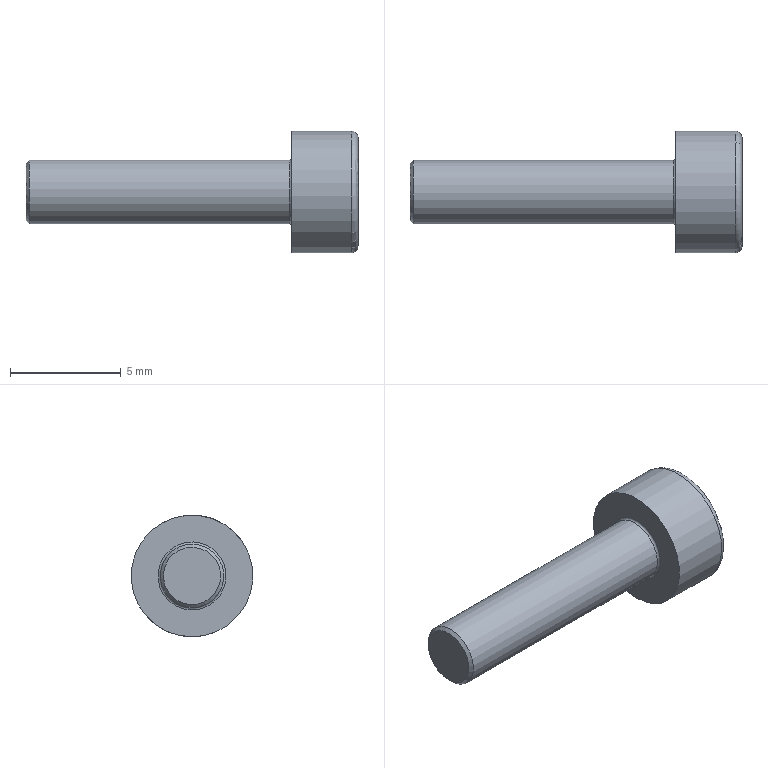Component | NX | GB-T70_1-2000_M3X12_2 | 1 solid | 27 faces | volume 137 mm3 | plane 15 | cone 8 | cylinder 2 | torus 2 | commonest cylinder face diameters 2.874 x1 5.5 x1